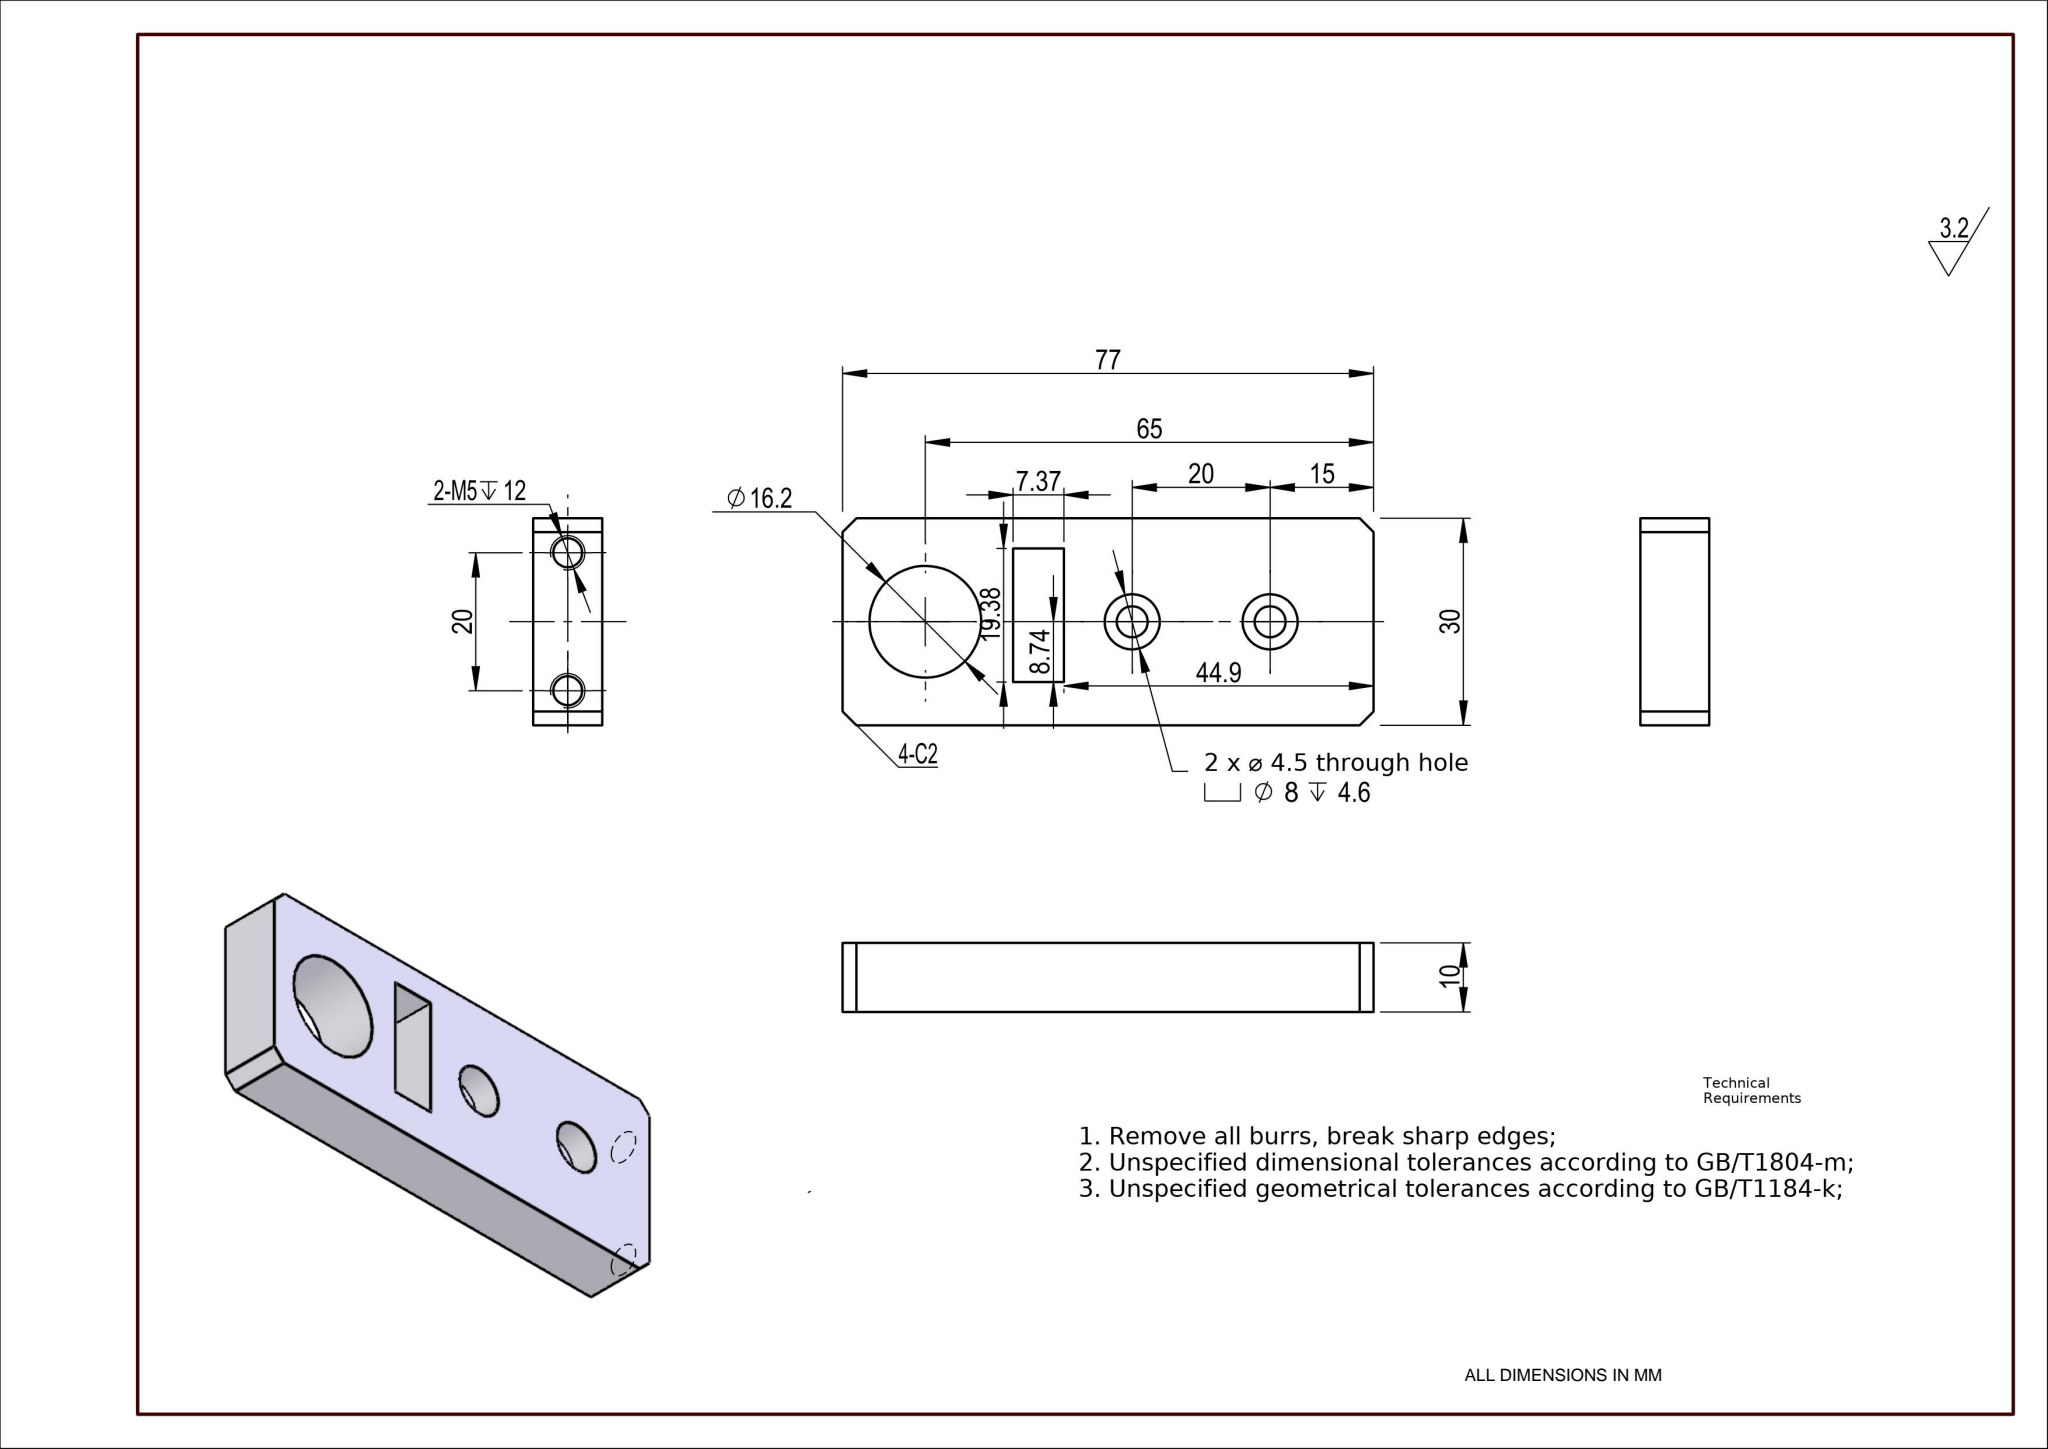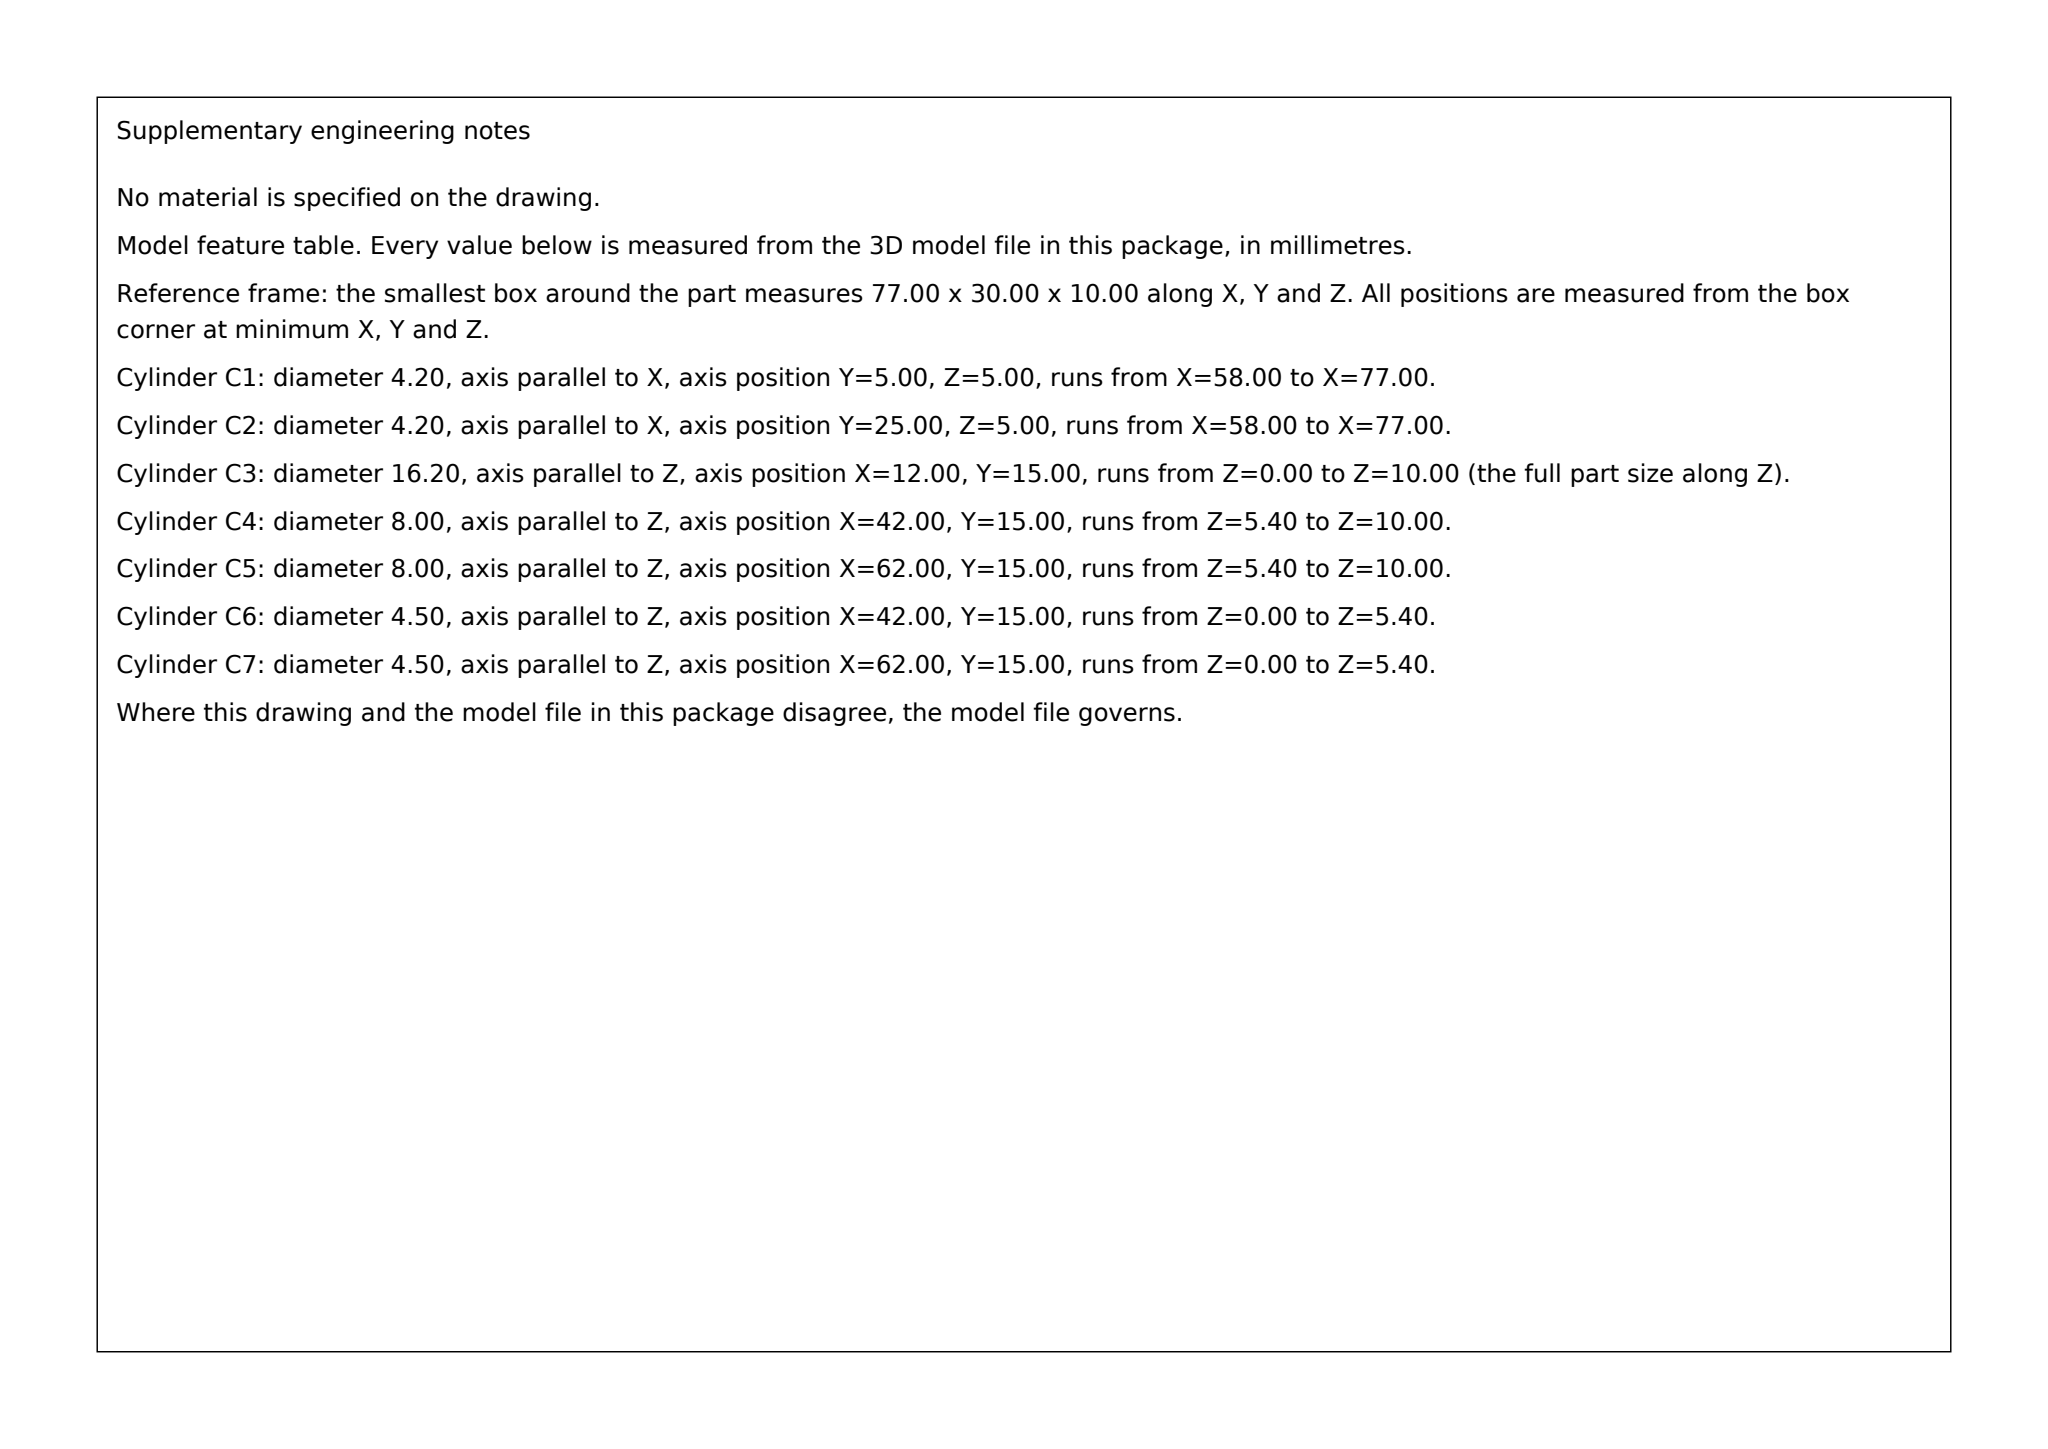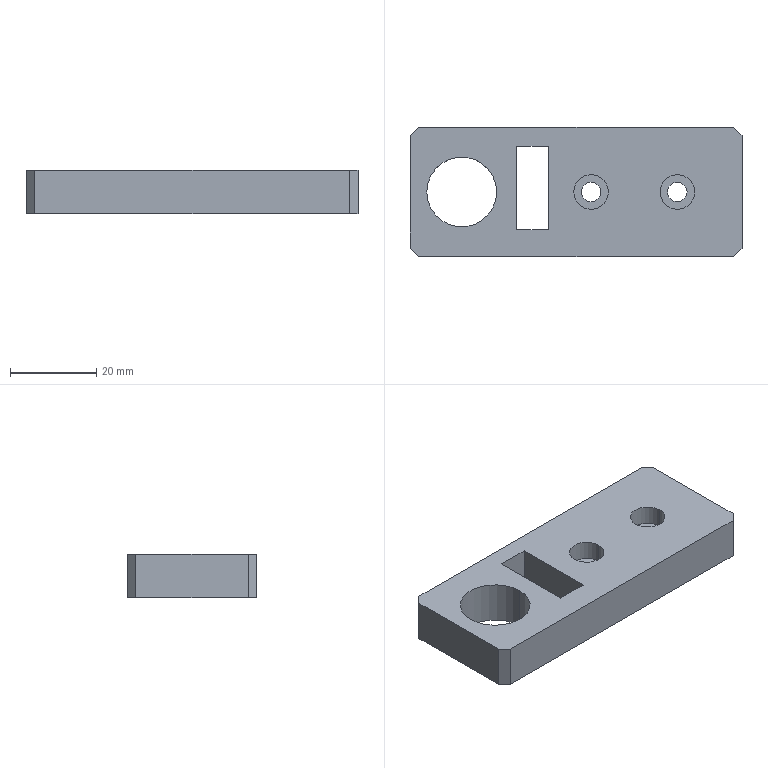Part | SolidWorks | mm | 1 solid | 34 faces | box 77 x 30 x 10 mm | volume 18358 mm3 | plane 16 | cylinder 14 | cone 4 | commonest cylinder face diameters 4.2 x4 8 x4 4.5 x4 16.2 x2
build123d program:
from build123d import *

# Parameters (mm, degrees)
SKETCH1_W                                            = 77
SKETCH1_H                                            = 30
BOSS_EXTRUDE1_DEPTH                                  = 5
HOLE_SIZE_ACCORDING_TO_HEX_SOCKET_HEAD_C_D           = 4.5
HOLE_SIZE_ACCORDING_TO_HEX_SOCKET_HEAD_C_CBORE_D     = 8
HOLE_SIZE_ACCORDING_TO_HEX_SOCKET_HEAD_C_CBORE_DEPTH = 4.6
SKETCH4_R                                            = 8.1
CUT_EXTRUDE1_DEPTH                                   = 43.512
M5_TAPPED_HOLE1_D                                    = 4.2
M5_TAPPED_HOLE1_DEPTH                                = 19
M5_TAPPED_HOLE1_TIP                                  = 1.262
CHAMFER1_SIZE                                        = 2
SKETCH7_W                                            = 7.372
SKETCH7_H                                            = 19.375
CUT_EXTRUDE2_DEPTH                                   = 31


with BuildPart() as part:
    # Sketch1 → Boss-Extrude1 (new, symmetric)
    with BuildSketch(Plane.XY):
        Rectangle(SKETCH1_W, SKETCH1_H)
    extrude(amount=BOSS_EXTRUDE1_DEPTH, both=True)

    # Hole size according to hex socket head c (through all)
    with Locations(Plane.XY.offset(5)):
        with Locations((3.5, 0), (23.5, 0)):
            CounterBoreHole(HOLE_SIZE_ACCORDING_TO_HEX_SOCKET_HEAD_C_D / 2, HOLE_SIZE_ACCORDING_TO_HEX_SOCKET_HEAD_C_CBORE_D / 2, HOLE_SIZE_ACCORDING_TO_HEX_SOCKET_HEAD_C_CBORE_DEPTH)

    # Sketch4 → Cut-Extrude1 (cut, through all)
    with BuildSketch(Plane.XY.offset(5)):
        with Locations((-26.5, 0)):
            Circle(SKETCH4_R)
    extrude(amount=-CUT_EXTRUDE1_DEPTH, mode=Mode.SUBTRACT)

    # M5 Tapped Hole1
    with Locations(Plane(origin=(38.5, 0, 0), x_dir=(0, 0, -1), z_dir=(1, 0, 0))):
        with Locations((0, 10), (0, -10)):
            Hole(M5_TAPPED_HOLE1_D / 2, depth=M5_TAPPED_HOLE1_DEPTH)
            with Locations((0, 0, -(M5_TAPPED_HOLE1_DEPTH + M5_TAPPED_HOLE1_TIP / 2))):  # 118° drill point
                Cone(0, M5_TAPPED_HOLE1_D / 2, M5_TAPPED_HOLE1_TIP, mode=Mode.SUBTRACT)

    # Chamfer1
    chamfer1_edges = [part.edges().sort_by_distance(p)[0] for p in [
        (38.5, -15, 0),
        (-38.5, -15, 0),
        (-38.5, 15, 0),
        (38.5, 15, 0),
    ]]
    chamfer(chamfer1_edges, length=CHAMFER1_SIZE)

    # Sketch7 → Cut-Extrude2 (cut)
    with BuildSketch(Plane.XY.offset(5)):
        with Locations((-10.084, 0.9444)):
            Rectangle(SKETCH7_W, SKETCH7_H)
    extrude(amount=-CUT_EXTRUDE2_DEPTH, mode=Mode.SUBTRACT)


solid = part.part